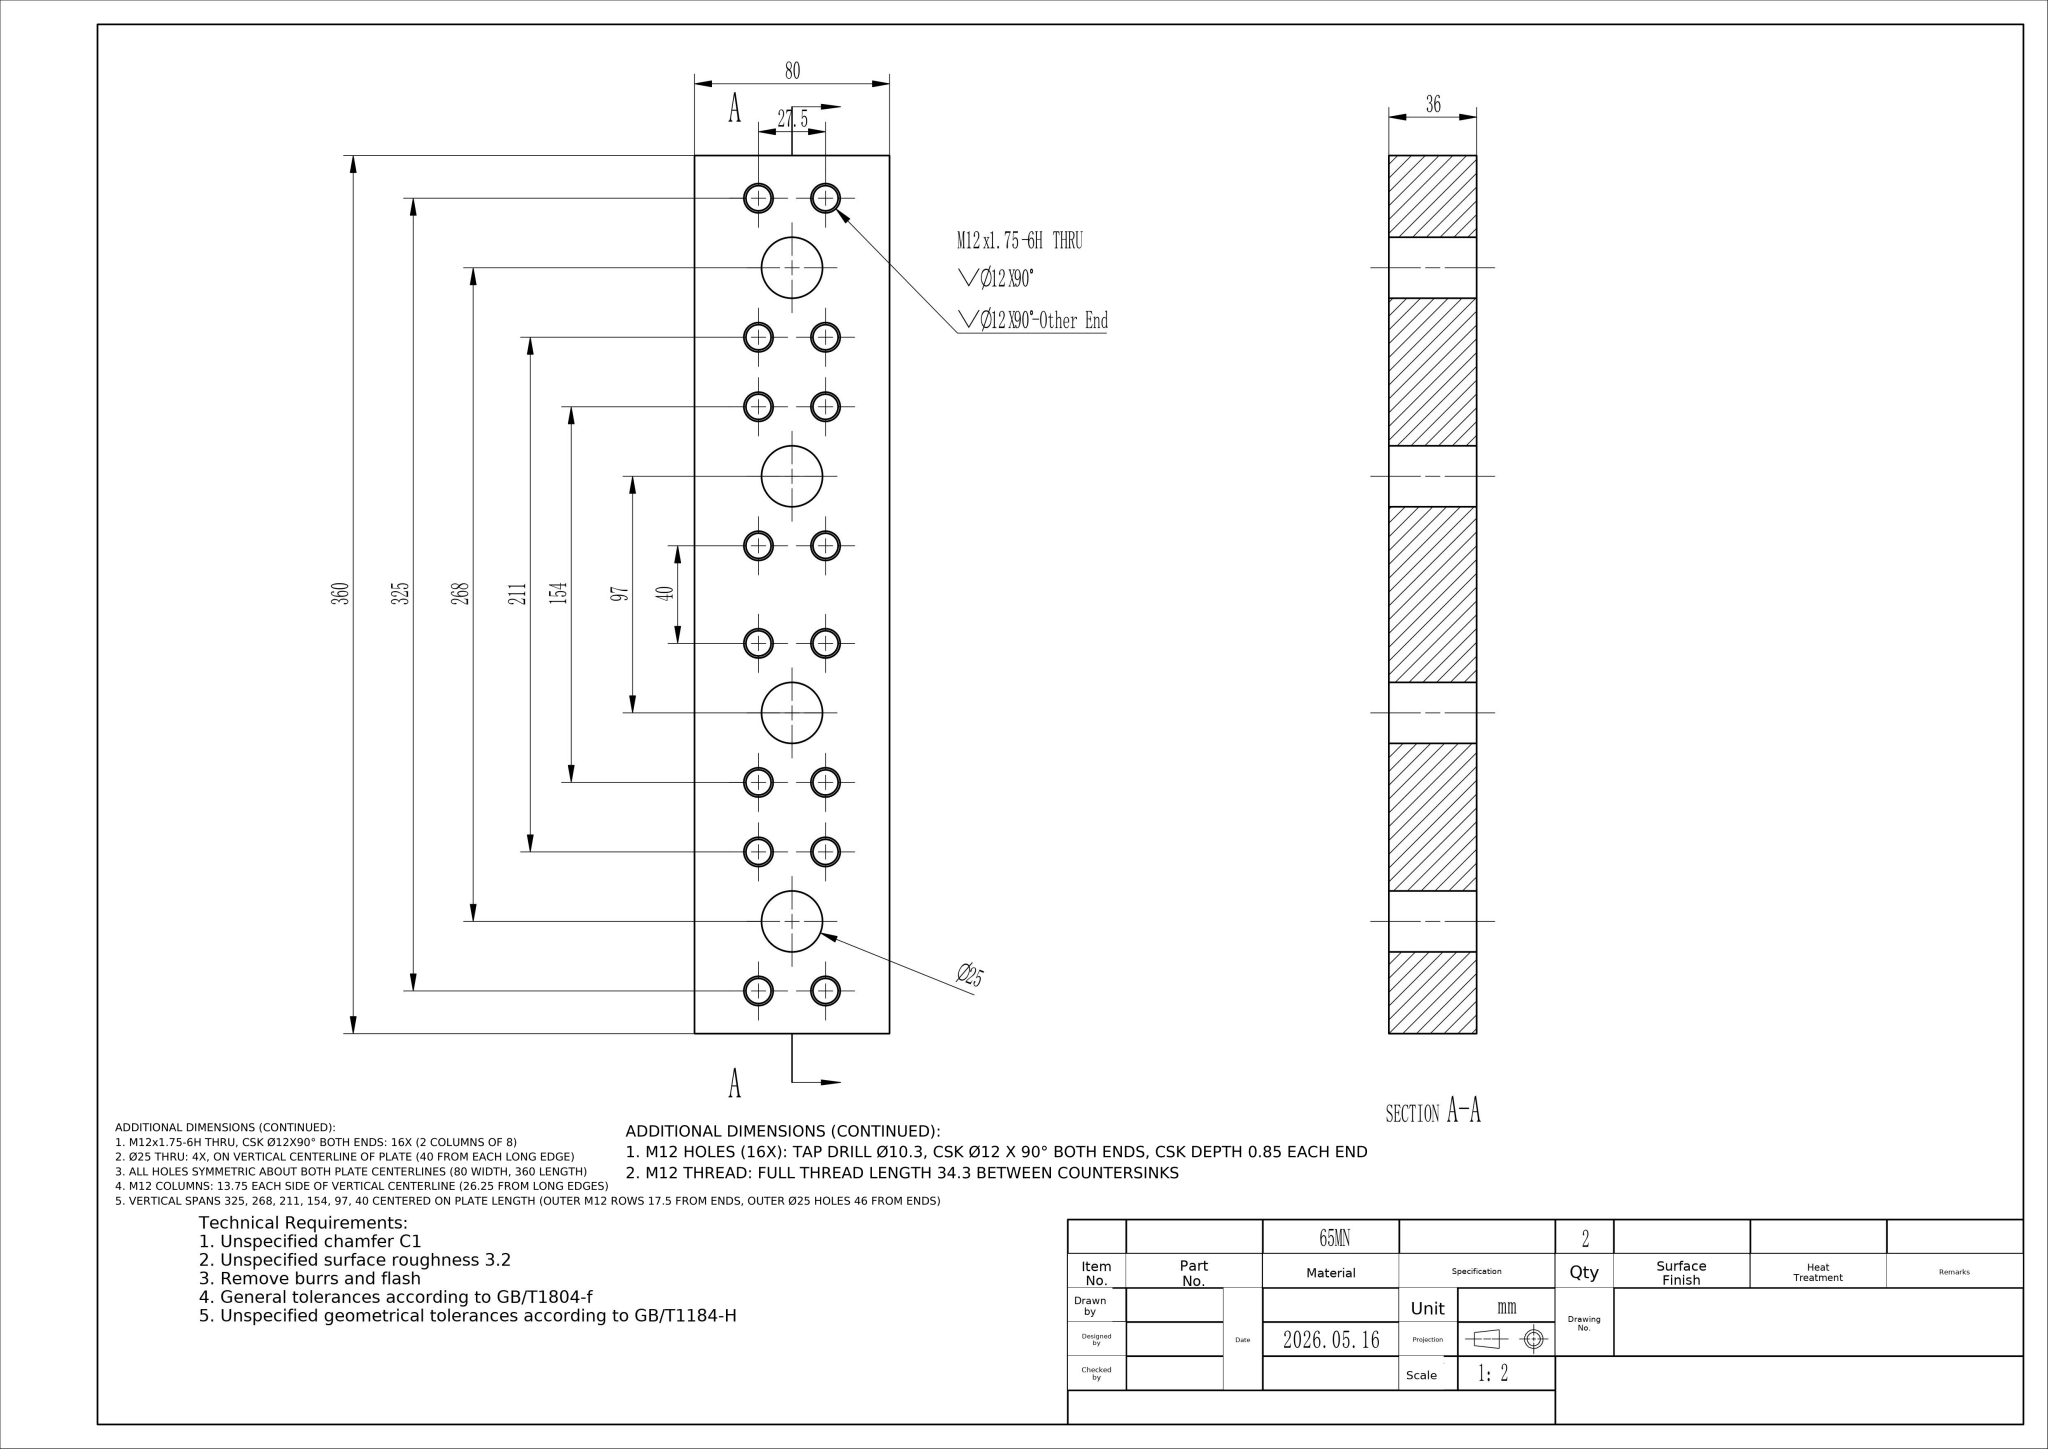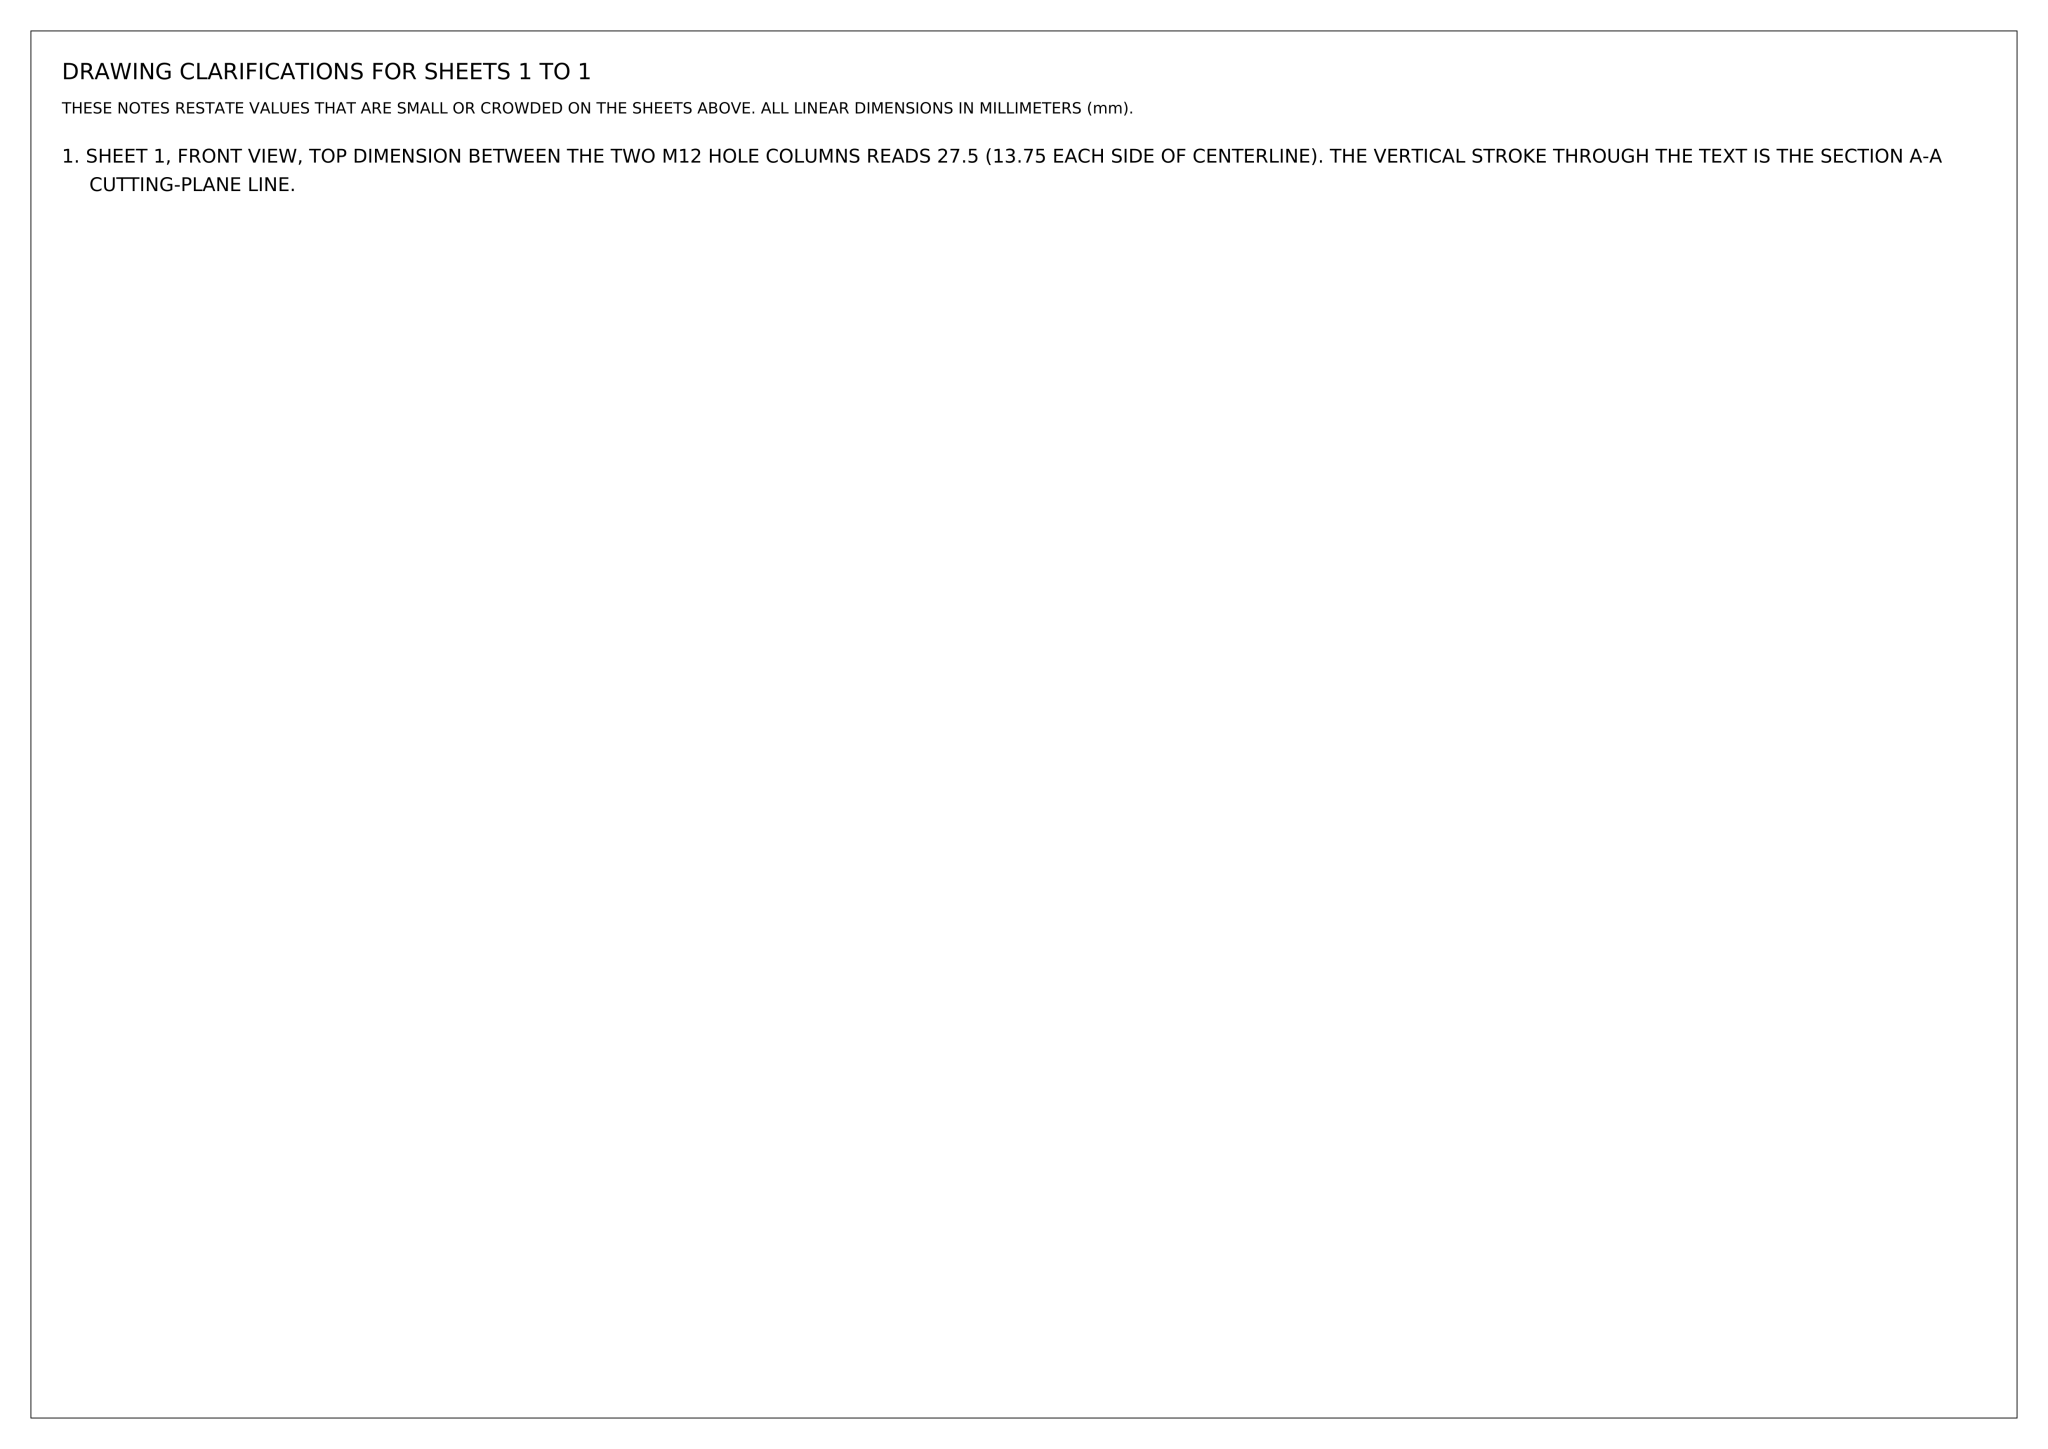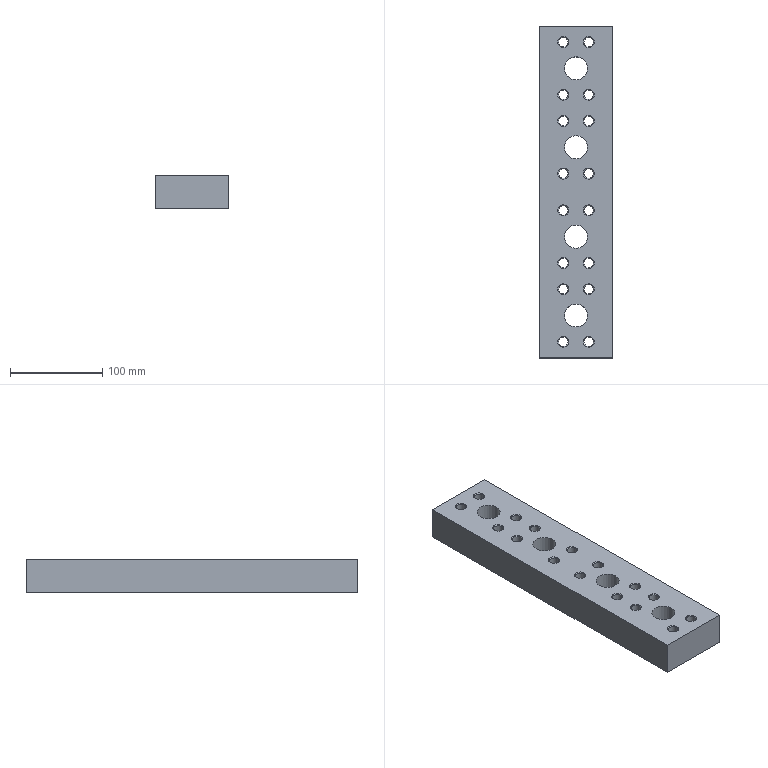Part | NX | mm | 1 solid | 58 faces | box 80 x 360 x 36 mm | volume 917726 mm3 | cone 32 | cylinder 20 | plane 6 | commonest cylinder face diameters 10.3 x16 25 x4